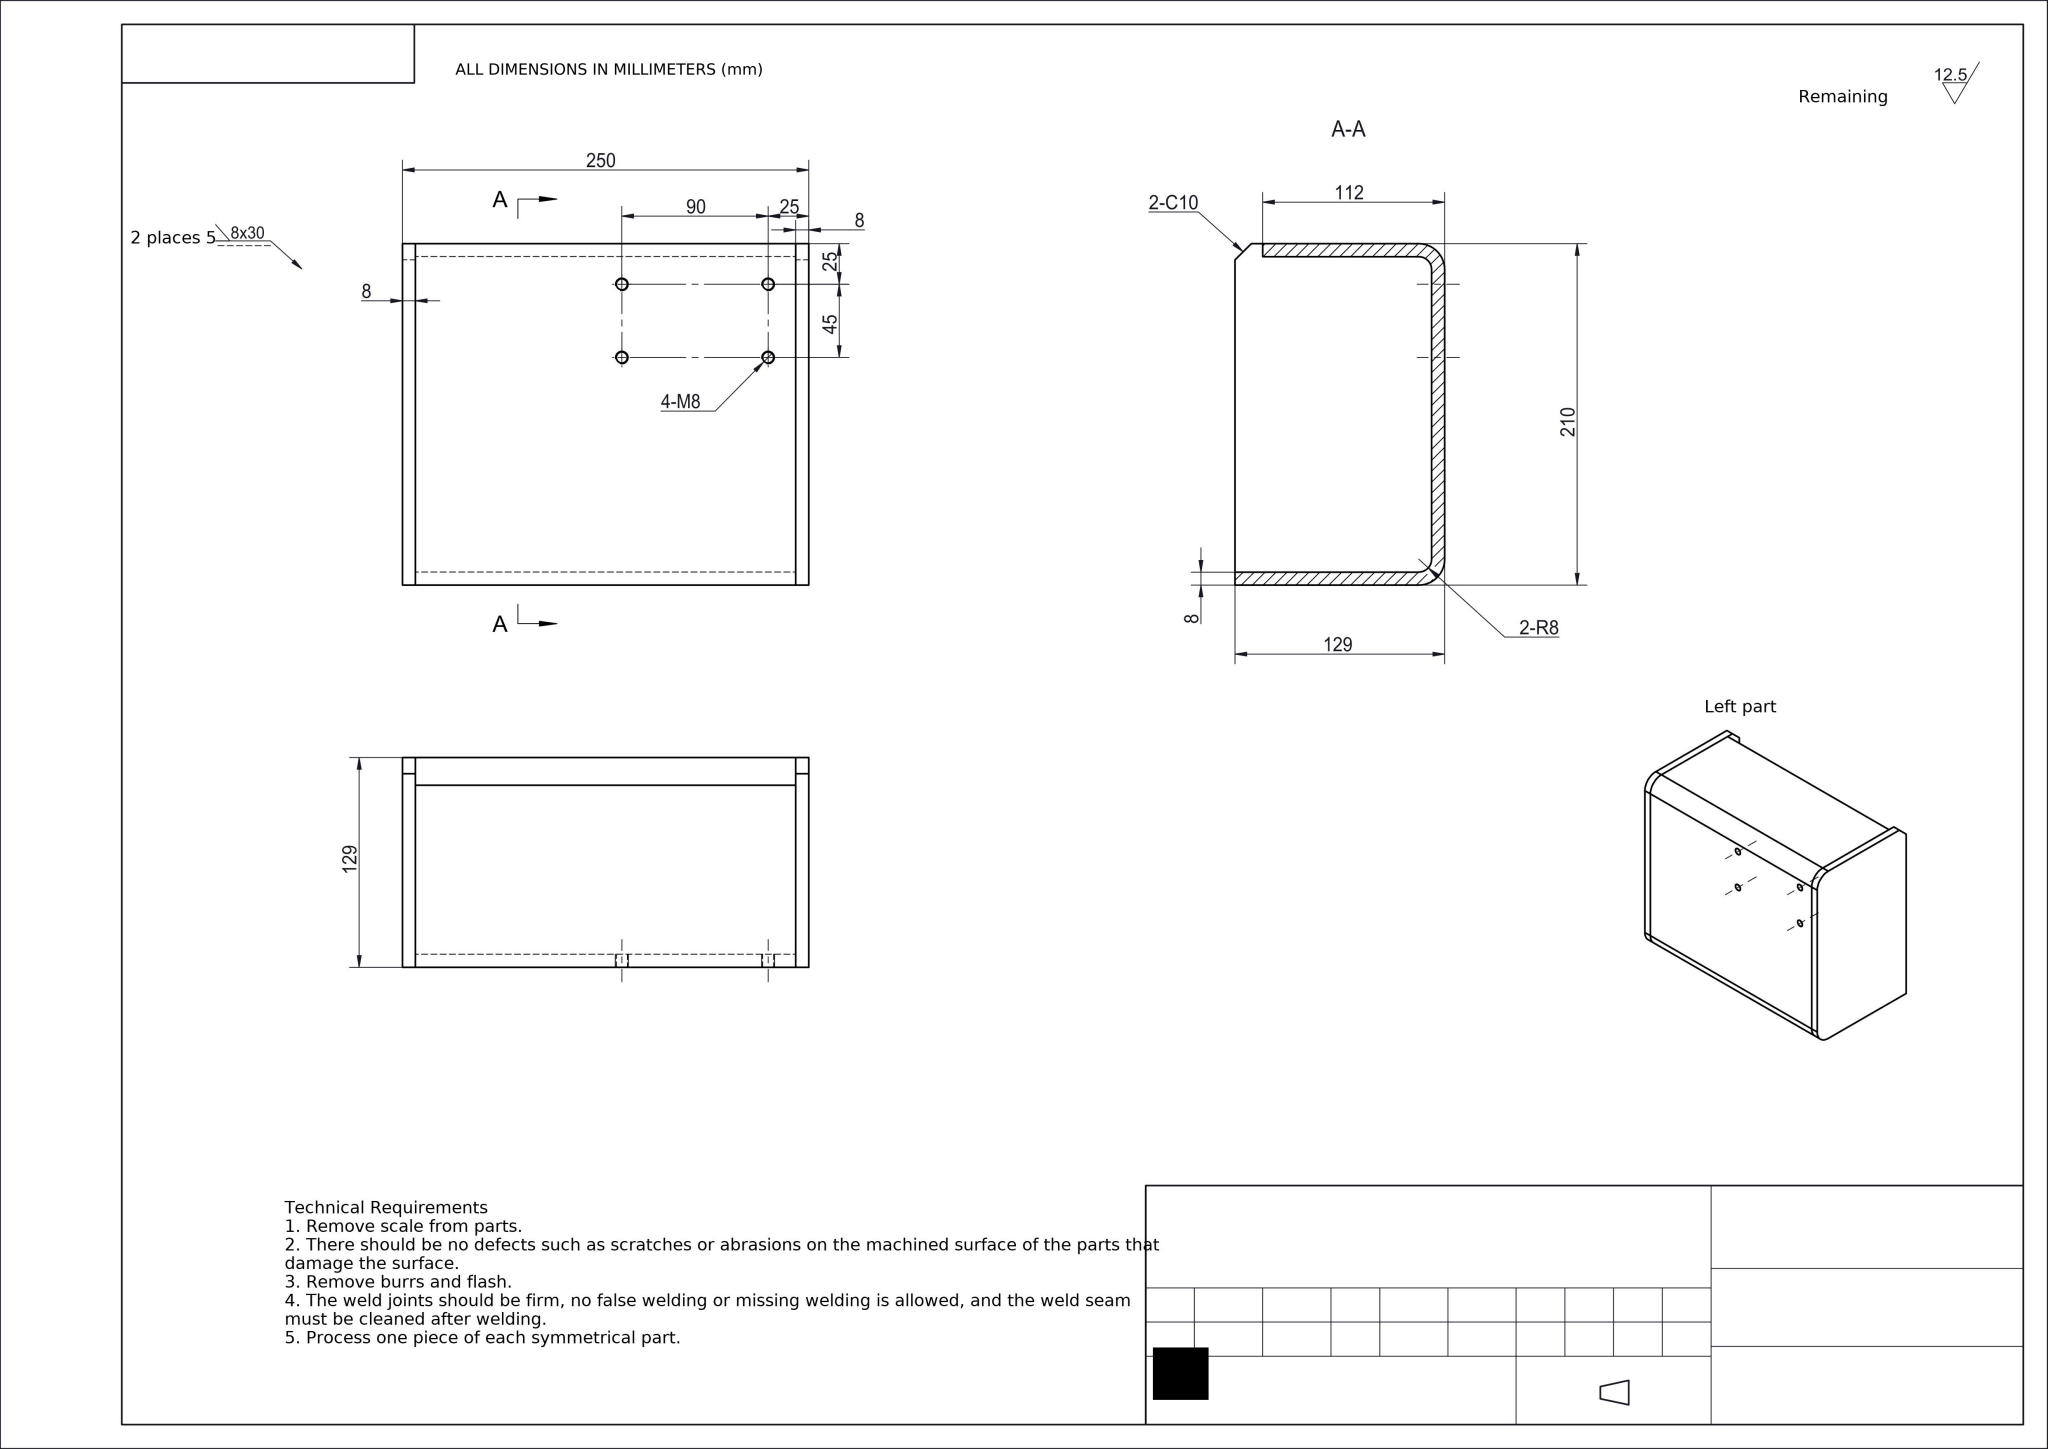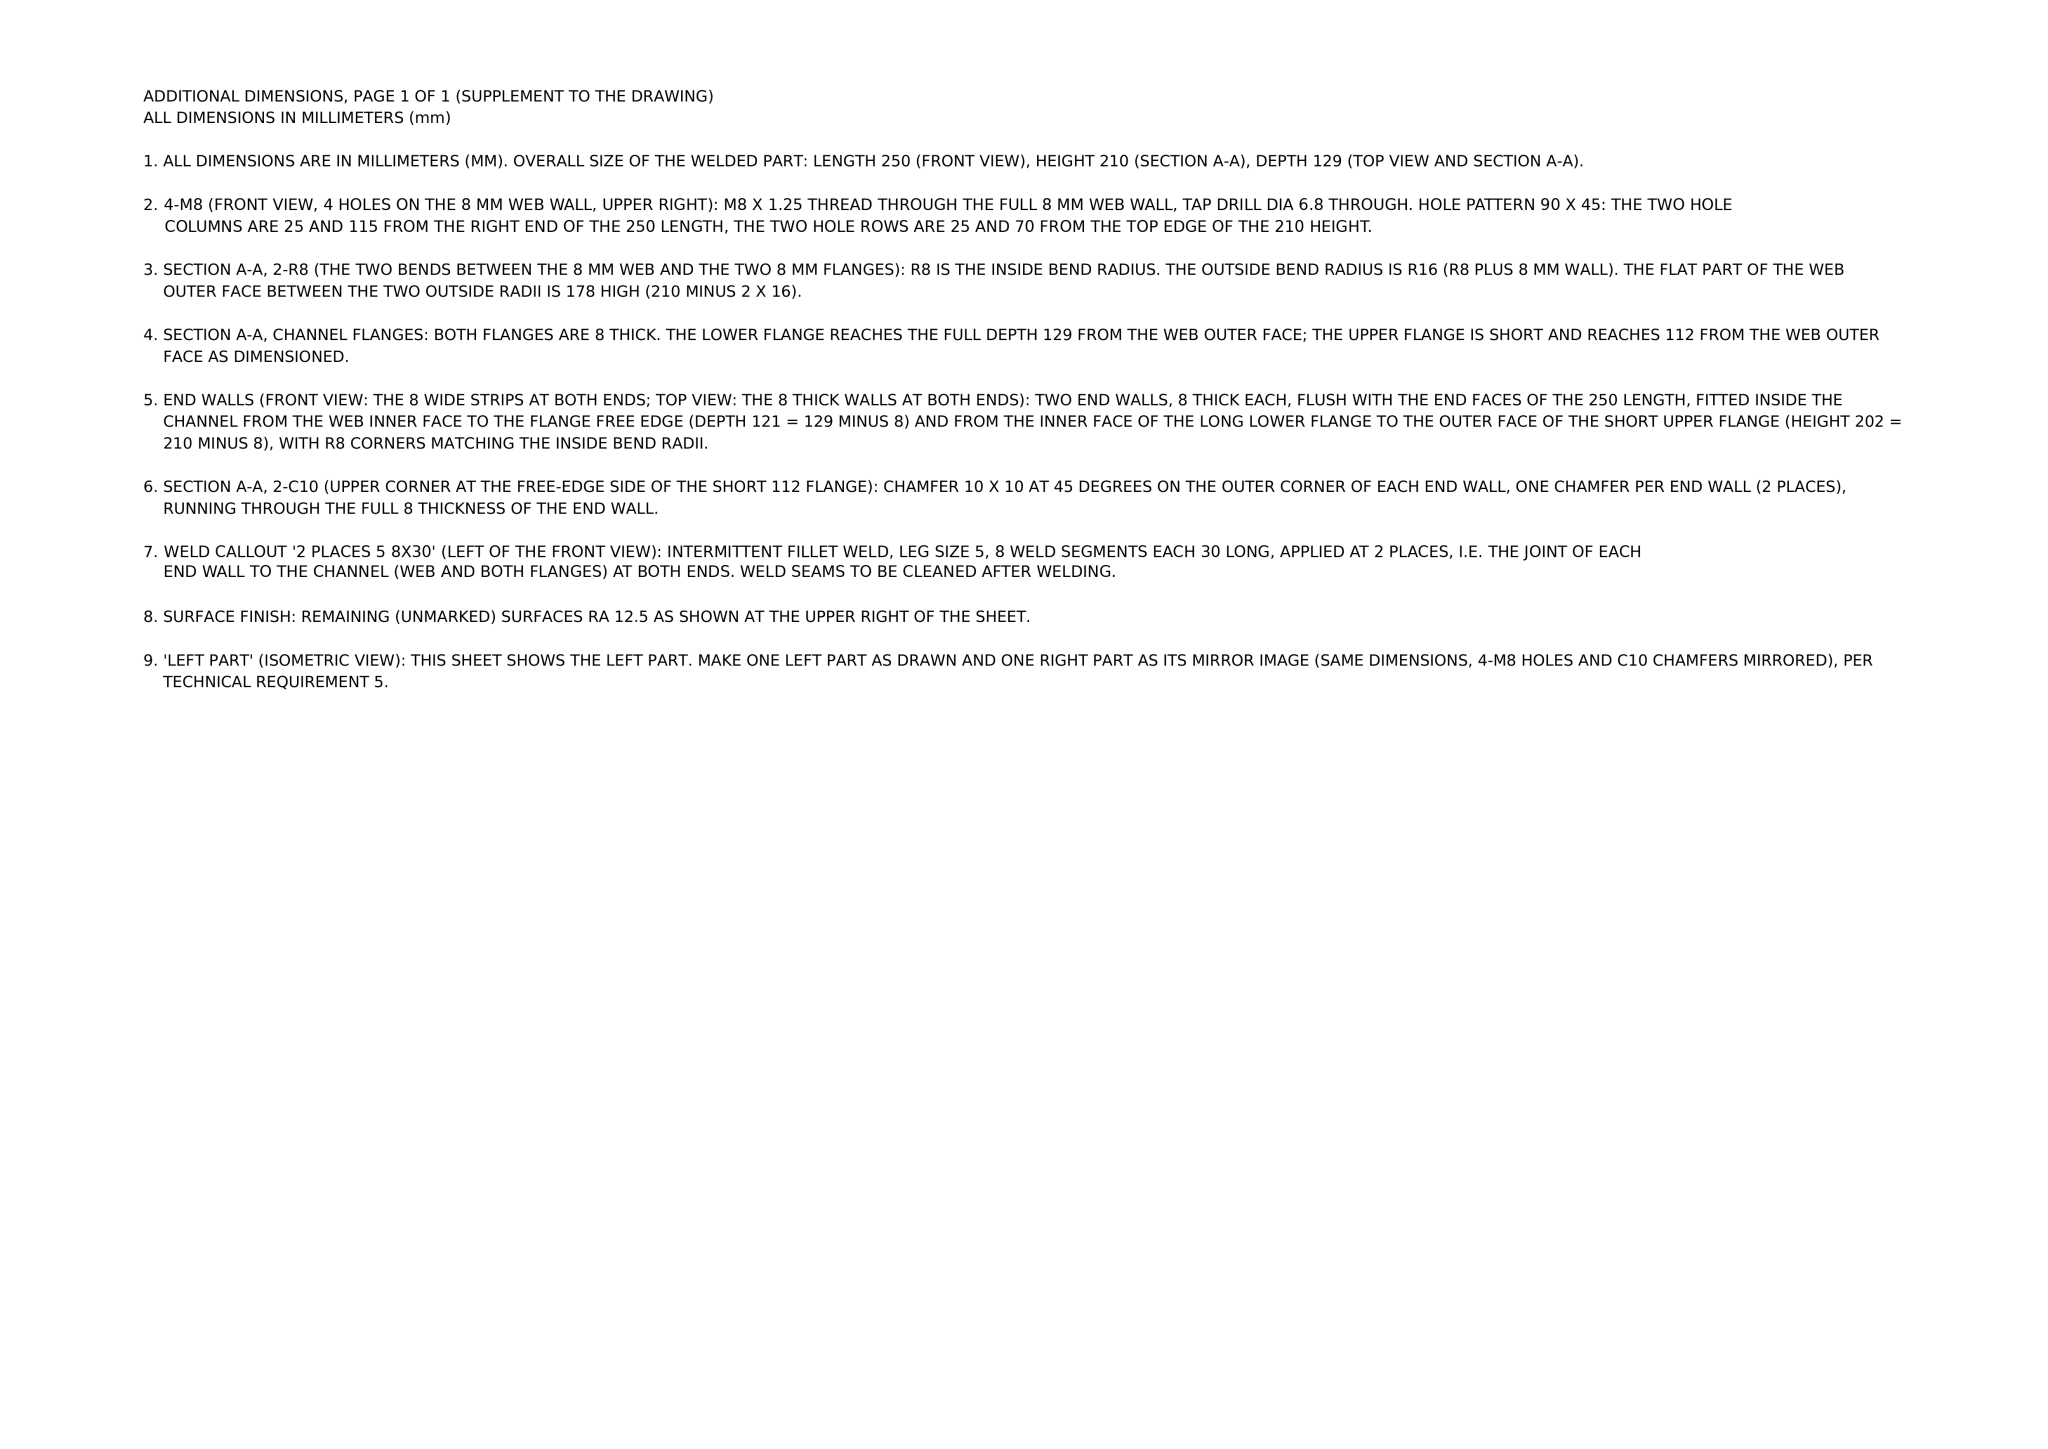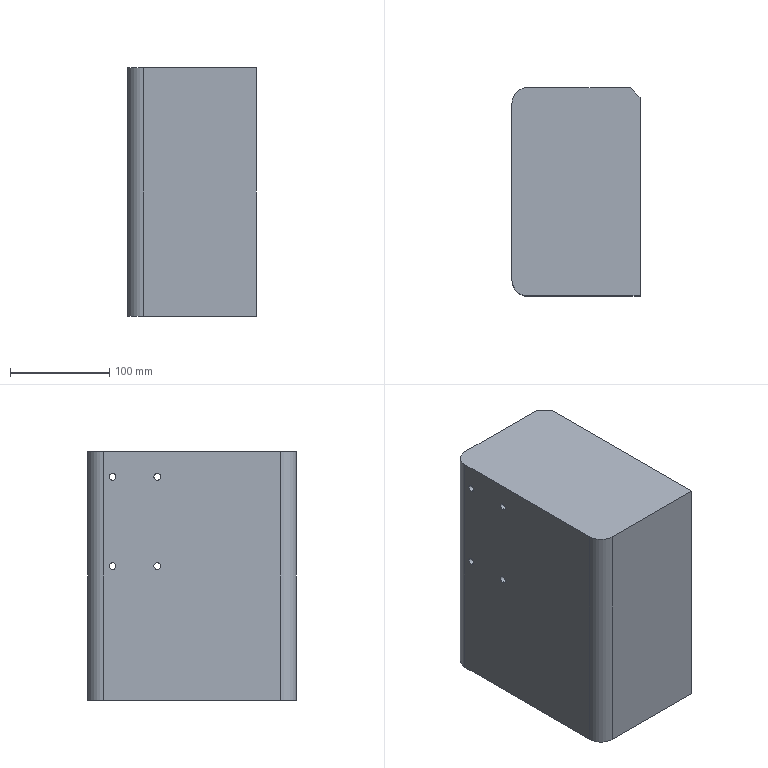Part | NX | mm | 1 solid | 26 faces | box 129 x 210 x 250 mm | volume 1224757 mm3 | plane 14 | cylinder 12 | commonest cylinder face diameters 6.8 x8 32 x2 16 x2
STEP:
#1=COLOUR_RGB('',0.7922,0.8196,0.9333);
#2=FILL_AREA_STYLE_COLOUR('',#1);
#3=FILL_AREA_STYLE('',(#2));
#4=SURFACE_STYLE_FILL_AREA(#3);
#5=SURFACE_SIDE_STYLE('',(#4));
#6=SURFACE_STYLE_USAGE(.BOTH.,#5);
#7=PRESENTATION_STYLE_ASSIGNMENT((#6));
#8=CARTESIAN_POINT('',(8.,80.,6.6));
#9=VERTEX_POINT('',#8);
#10=CARTESIAN_POINT('',(0.,80.,6.6));
#11=VERTEX_POINT('',#10);
#12=CARTESIAN_POINT('',(0.,80.,6.6));
#13=DIRECTION('',(-1.,0.,0.));
#14=VECTOR('',#13,1000.);
#15=LINE('',#12,#14);
#16=EDGE_CURVE('',#9,#11,#15,.T.);
#17=ORIENTED_EDGE('',*,*,#16,.F.);
#18=CARTESIAN_POINT('',(8.,80.,13.4));
#19=VERTEX_POINT('',#18);
#20=CARTESIAN_POINT('',(8.,80.,10.));
#21=DIRECTION('',(1.,0.,0.));
#22=DIRECTION('',(0.,1.,0.));
#23=AXIS2_PLACEMENT_3D('',#20,#21,#22);
#24=CIRCLE('',#23,3.4);
#25=EDGE_CURVE('',#9,#19,#24,.T.);
#26=ORIENTED_EDGE('',*,*,#25,.T.);
#27=CARTESIAN_POINT('',(0.,80.,13.4));
#28=VERTEX_POINT('',#27);
#29=CARTESIAN_POINT('',(0.,80.,13.4));
#30=DIRECTION('',(-1.,0.,0.));
#31=VECTOR('',#30,1000.);
#32=LINE('',#29,#31);
#33=EDGE_CURVE('',#19,#28,#32,.T.);
#34=ORIENTED_EDGE('',*,*,#33,.T.);
#35=CARTESIAN_POINT('',(0.,80.,10.));
#36=DIRECTION('',(-1.,0.,0.));
#37=DIRECTION('',(0.,0.,1.));
#38=AXIS2_PLACEMENT_3D('',#35,#36,#37);
#39=CIRCLE('',#38,3.4);
#40=EDGE_CURVE('',#28,#11,#39,.T.);
#41=ORIENTED_EDGE('',*,*,#40,.T.);
#42=EDGE_LOOP('',(#17,#26,#34,#41));
#43=FACE_OUTER_BOUND('',#42,.T.);
#44=CARTESIAN_POINT('',(0.,80.,10.));
#45=DIRECTION('',(-1.,0.,0.));
#46=DIRECTION('',(0.,0.,1.));
#47=AXIS2_PLACEMENT_3D('',#44,#45,#46);
#48=CYLINDRICAL_SURFACE('',#47,3.4);
#49=ADVANCED_FACE('',(#43),#48,.F.);
#50=CARTESIAN_POINT('',(8.,35.,6.6));
#51=VERTEX_POINT('',#50);
#52=CARTESIAN_POINT('',(-0.,35.,6.6));
#53=VERTEX_POINT('',#52);
#54=CARTESIAN_POINT('',(-0.,35.,6.6));
#55=DIRECTION('',(-1.,0.,0.));
#56=VECTOR('',#55,1000.);
#57=LINE('',#54,#56);
#58=EDGE_CURVE('',#51,#53,#57,.T.);
#59=ORIENTED_EDGE('',*,*,#58,.F.);
#60=CARTESIAN_POINT('',(8.,35.,13.4));
#61=VERTEX_POINT('',#60);
#62=CARTESIAN_POINT('',(8.,35.,10.));
#63=DIRECTION('',(1.,0.,0.));
#64=DIRECTION('',(0.,1.,0.));
#65=AXIS2_PLACEMENT_3D('',#62,#63,#64);
#66=CIRCLE('',#65,3.4);
#67=EDGE_CURVE('',#51,#61,#66,.T.);
#68=ORIENTED_EDGE('',*,*,#67,.T.);
#69=CARTESIAN_POINT('',(-0.,35.,13.4));
#70=VERTEX_POINT('',#69);
#71=CARTESIAN_POINT('',(-0.,35.,13.4));
#72=DIRECTION('',(-1.,0.,0.));
#73=VECTOR('',#72,1000.);
#74=LINE('',#71,#73);
#75=EDGE_CURVE('',#61,#70,#74,.T.);
#76=ORIENTED_EDGE('',*,*,#75,.T.);
#77=CARTESIAN_POINT('',(-0.,35.,10.));
#78=DIRECTION('',(-1.,0.,0.));
#79=DIRECTION('',(0.,0.,1.));
#80=AXIS2_PLACEMENT_3D('',#77,#78,#79);
#81=CIRCLE('',#80,3.4);
#82=EDGE_CURVE('',#70,#53,#81,.T.);
#83=ORIENTED_EDGE('',*,*,#82,.T.);
#84=EDGE_LOOP('',(#59,#68,#76,#83));
#85=FACE_OUTER_BOUND('',#84,.T.);
#86=CARTESIAN_POINT('',(-0.,35.,10.));
#87=DIRECTION('',(-1.,0.,0.));
#88=DIRECTION('',(0.,0.,1.));
#89=AXIS2_PLACEMENT_3D('',#86,#87,#88);
#90=CYLINDRICAL_SURFACE('',#89,3.4);
#91=ADVANCED_FACE('',(#85),#90,.F.);
#92=CARTESIAN_POINT('',(8.,80.,96.6));
#93=VERTEX_POINT('',#92);
#94=CARTESIAN_POINT('',(0.,80.,96.6));
#95=VERTEX_POINT('',#94);
#96=CARTESIAN_POINT('',(0.,80.,96.6));
#97=DIRECTION('',(-1.,0.,0.));
#98=VECTOR('',#97,1000.);
#99=LINE('',#96,#98);
#100=EDGE_CURVE('',#93,#95,#99,.T.);
#101=ORIENTED_EDGE('',*,*,#100,.F.);
#102=CARTESIAN_POINT('',(8.,80.,103.4));
#103=VERTEX_POINT('',#102);
#104=CARTESIAN_POINT('',(8.,80.,100.));
#105=DIRECTION('',(1.,0.,0.));
#106=DIRECTION('',(0.,1.,0.));
#107=AXIS2_PLACEMENT_3D('',#104,#105,#106);
#108=CIRCLE('',#107,3.4);
#109=EDGE_CURVE('',#93,#103,#108,.T.);
#110=ORIENTED_EDGE('',*,*,#109,.T.);
#111=CARTESIAN_POINT('',(0.,80.,103.4));
#112=VERTEX_POINT('',#111);
#113=CARTESIAN_POINT('',(0.,80.,103.4));
#114=DIRECTION('',(-1.,0.,0.));
#115=VECTOR('',#114,1000.);
#116=LINE('',#113,#115);
#117=EDGE_CURVE('',#103,#112,#116,.T.);
#118=ORIENTED_EDGE('',*,*,#117,.T.);
#119=CARTESIAN_POINT('',(0.,80.,100.));
#120=DIRECTION('',(-1.,0.,0.));
#121=DIRECTION('',(0.,0.,1.));
#122=AXIS2_PLACEMENT_3D('',#119,#120,#121);
#123=CIRCLE('',#122,3.4);
#124=EDGE_CURVE('',#112,#95,#123,.T.);
#125=ORIENTED_EDGE('',*,*,#124,.T.);
#126=EDGE_LOOP('',(#101,#110,#118,#125));
#127=FACE_OUTER_BOUND('',#126,.T.);
#128=CARTESIAN_POINT('',(0.,80.,100.));
#129=DIRECTION('',(-1.,0.,0.));
#130=DIRECTION('',(0.,0.,1.));
#131=AXIS2_PLACEMENT_3D('',#128,#129,#130);
#132=CYLINDRICAL_SURFACE('',#131,3.4);
#133=ADVANCED_FACE('',(#127),#132,.F.);
#134=CARTESIAN_POINT('',(8.,35.,96.6));
#135=VERTEX_POINT('',#134);
#136=CARTESIAN_POINT('',(-0.,35.,96.6));
#137=VERTEX_POINT('',#136);
#138=CARTESIAN_POINT('',(-0.,35.,96.6));
#139=DIRECTION('',(-1.,0.,0.));
#140=VECTOR('',#139,1000.);
#141=LINE('',#138,#140);
#142=EDGE_CURVE('',#135,#137,#141,.T.);
#143=ORIENTED_EDGE('',*,*,#142,.F.);
#144=CARTESIAN_POINT('',(8.,35.,103.4));
#145=VERTEX_POINT('',#144);
#146=CARTESIAN_POINT('',(8.,35.,100.));
#147=DIRECTION('',(1.,0.,0.));
#148=DIRECTION('',(0.,1.,0.));
#149=AXIS2_PLACEMENT_3D('',#146,#147,#148);
#150=CIRCLE('',#149,3.4);
#151=EDGE_CURVE('',#135,#145,#150,.T.);
#152=ORIENTED_EDGE('',*,*,#151,.T.);
#153=CARTESIAN_POINT('',(-0.,35.,103.4));
#154=VERTEX_POINT('',#153);
#155=CARTESIAN_POINT('',(-0.,35.,103.4));
#156=DIRECTION('',(-1.,0.,0.));
#157=VECTOR('',#156,1000.);
#158=LINE('',#155,#157);
#159=EDGE_CURVE('',#145,#154,#158,.T.);
#160=ORIENTED_EDGE('',*,*,#159,.T.);
#161=CARTESIAN_POINT('',(-0.,35.,100.));
#162=DIRECTION('',(-1.,0.,0.));
#163=DIRECTION('',(0.,0.,1.));
#164=AXIS2_PLACEMENT_3D('',#161,#162,#163);
#165=CIRCLE('',#164,3.4);
#166=EDGE_CURVE('',#154,#137,#165,.T.);
#167=ORIENTED_EDGE('',*,*,#166,.T.);
#168=EDGE_LOOP('',(#143,#152,#160,#167));
#169=FACE_OUTER_BOUND('',#168,.T.);
#170=CARTESIAN_POINT('',(-0.,35.,100.));
#171=DIRECTION('',(-1.,0.,0.));
#172=DIRECTION('',(0.,0.,1.));
#173=AXIS2_PLACEMENT_3D('',#170,#171,#172);
#174=CYLINDRICAL_SURFACE('',#173,3.4);
#175=ADVANCED_FACE('',(#169),#174,.F.);
#176=CARTESIAN_POINT('',(-0.,-89.,125.));
#177=VERTEX_POINT('',#176);
#178=CARTESIAN_POINT('',(-0.,-89.,-125.));
#179=VERTEX_POINT('',#178);
#180=CARTESIAN_POINT('',(-0.,-89.,117.));
#181=DIRECTION('',(0.,0.,-1.));
#182=VECTOR('',#181,1000.);
#183=LINE('',#180,#182);
#184=EDGE_CURVE('',#177,#179,#183,.T.);
#185=ORIENTED_EDGE('',*,*,#184,.T.);
#186=CARTESIAN_POINT('',(16.,-105.,-125.));
#187=VERTEX_POINT('',#186);
#188=CARTESIAN_POINT('',(16.,-89.,-125.));
#189=DIRECTION('',(0.,-0.,-1.));
#190=DIRECTION('',(-1.,0.,0.));
#191=AXIS2_PLACEMENT_3D('',#188,#189,#190);
#192=CIRCLE('',#191,16.);
#193=EDGE_CURVE('',#187,#179,#192,.T.);
#194=ORIENTED_EDGE('',*,*,#193,.F.);
#195=CARTESIAN_POINT('',(16.,-105.,125.));
#196=VERTEX_POINT('',#195);
#197=CARTESIAN_POINT('',(16.,-105.,117.));
#198=DIRECTION('',(0.,0.,-1.));
#199=VECTOR('',#198,1000.);
#200=LINE('',#197,#199);
#201=EDGE_CURVE('',#196,#187,#200,.T.);
#202=ORIENTED_EDGE('',*,*,#201,.F.);
#203=CARTESIAN_POINT('',(16.,-89.,125.));
#204=DIRECTION('',(0.,0.,1.));
#205=DIRECTION('',(1.,0.,0.));
#206=AXIS2_PLACEMENT_3D('',#203,#204,#205);
#207=CIRCLE('',#206,16.);
#208=EDGE_CURVE('',#177,#196,#207,.T.);
#209=ORIENTED_EDGE('',*,*,#208,.F.);
#210=EDGE_LOOP('',(#185,#194,#202,#209));
#211=FACE_OUTER_BOUND('',#210,.T.);
#212=CARTESIAN_POINT('',(16.,-89.,117.));
#213=DIRECTION('',(0.,0.,-1.));
#214=DIRECTION('',(-1.,0.,0.));
#215=AXIS2_PLACEMENT_3D('',#212,#213,#214);
#216=CYLINDRICAL_SURFACE('',#215,16.);
#217=ADVANCED_FACE('',(#211),#216,.T.);
#218=ORIENTED_EDGE('',*,*,#166,.F.);
#219=CARTESIAN_POINT('',(-0.,35.,100.));
#220=DIRECTION('',(-1.,0.,0.));
#221=DIRECTION('',(0.,0.,1.));
#222=AXIS2_PLACEMENT_3D('',#219,#220,#221);
#223=CIRCLE('',#222,3.4);
#224=EDGE_CURVE('',#137,#154,#223,.T.);
#225=ORIENTED_EDGE('',*,*,#224,.F.);
#226=EDGE_LOOP('',(#218,#225));
#227=FACE_BOUND('',#226,.T.);
#228=ORIENTED_EDGE('',*,*,#124,.F.);
#229=CARTESIAN_POINT('',(0.,80.,100.));
#230=DIRECTION('',(-1.,0.,0.));
#231=DIRECTION('',(0.,0.,1.));
#232=AXIS2_PLACEMENT_3D('',#229,#230,#231);
#233=CIRCLE('',#232,3.4);
#234=EDGE_CURVE('',#95,#112,#233,.T.);
#235=ORIENTED_EDGE('',*,*,#234,.F.);
#236=EDGE_LOOP('',(#228,#235));
#237=FACE_BOUND('',#236,.T.);
#238=ORIENTED_EDGE('',*,*,#82,.F.);
#239=CARTESIAN_POINT('',(-0.,35.,10.));
#240=DIRECTION('',(-1.,0.,0.));
#241=DIRECTION('',(0.,0.,1.));
#242=AXIS2_PLACEMENT_3D('',#239,#240,#241);
#243=CIRCLE('',#242,3.4);
#244=EDGE_CURVE('',#53,#70,#243,.T.);
#245=ORIENTED_EDGE('',*,*,#244,.F.);
#246=EDGE_LOOP('',(#238,#245));
#247=FACE_BOUND('',#246,.T.);
#248=ORIENTED_EDGE('',*,*,#40,.F.);
#249=CARTESIAN_POINT('',(0.,80.,10.));
#250=DIRECTION('',(-1.,0.,0.));
#251=DIRECTION('',(0.,0.,1.));
#252=AXIS2_PLACEMENT_3D('',#249,#250,#251);
#253=CIRCLE('',#252,3.4);
#254=EDGE_CURVE('',#11,#28,#253,.T.);
#255=ORIENTED_EDGE('',*,*,#254,.F.);
#256=EDGE_LOOP('',(#248,#255));
#257=FACE_BOUND('',#256,.T.);
#258=CARTESIAN_POINT('',(0.,89.,125.));
#259=VERTEX_POINT('',#258);
#260=CARTESIAN_POINT('',(0.,89.,-125.));
#261=VERTEX_POINT('',#260);
#262=CARTESIAN_POINT('',(0.,89.,117.));
#263=DIRECTION('',(0.,0.,-1.));
#264=VECTOR('',#263,1000.);
#265=LINE('',#262,#264);
#266=EDGE_CURVE('',#259,#261,#265,.T.);
#267=ORIENTED_EDGE('',*,*,#266,.T.);
#268=CARTESIAN_POINT('',(-0.,105.,-125.));
#269=DIRECTION('',(-0.,-1.,-0.));
#270=VECTOR('',#269,1000.);
#271=LINE('',#268,#270);
#272=EDGE_CURVE('',#261,#179,#271,.T.);
#273=ORIENTED_EDGE('',*,*,#272,.T.);
#274=ORIENTED_EDGE('',*,*,#184,.F.);
#275=CARTESIAN_POINT('',(-0.,105.,125.));
#276=DIRECTION('',(0.,-1.,-0.));
#277=VECTOR('',#276,1000.);
#278=LINE('',#275,#277);
#279=EDGE_CURVE('',#259,#177,#278,.T.);
#280=ORIENTED_EDGE('',*,*,#279,.F.);
#281=EDGE_LOOP('',(#267,#273,#274,#280));
#282=FACE_OUTER_BOUND('',#281,.T.);
#283=CARTESIAN_POINT('',(-0.,105.,117.));
#284=DIRECTION('',(1.,0.,0.));
#285=DIRECTION('',(0.,1.,0.));
#286=AXIS2_PLACEMENT_3D('',#283,#284,#285);
#287=PLANE('',#286);
#288=ADVANCED_FACE('',(#227,#237,#247,#257,#282),#287,.F.);
#289=CARTESIAN_POINT('',(16.,105.,125.));
#290=VERTEX_POINT('',#289);
#291=CARTESIAN_POINT('',(16.,105.,-125.));
#292=VERTEX_POINT('',#291);
#293=CARTESIAN_POINT('',(16.,105.,117.));
#294=DIRECTION('',(0.,0.,-1.));
#295=VECTOR('',#294,1000.);
#296=LINE('',#293,#295);
#297=EDGE_CURVE('',#290,#292,#296,.T.);
#298=ORIENTED_EDGE('',*,*,#297,.T.);
#299=CARTESIAN_POINT('',(16.,89.,-125.));
#300=DIRECTION('',(0.,-0.,-1.));
#301=DIRECTION('',(-1.,0.,0.));
#302=AXIS2_PLACEMENT_3D('',#299,#300,#301);
#303=CIRCLE('',#302,16.);
#304=EDGE_CURVE('',#261,#292,#303,.T.);
#305=ORIENTED_EDGE('',*,*,#304,.F.);
#306=ORIENTED_EDGE('',*,*,#266,.F.);
#307=CARTESIAN_POINT('',(16.,89.,125.));
#308=DIRECTION('',(0.,0.,1.));
#309=DIRECTION('',(1.,0.,0.));
#310=AXIS2_PLACEMENT_3D('',#307,#308,#309);
#311=CIRCLE('',#310,16.);
#312=EDGE_CURVE('',#290,#259,#311,.T.);
#313=ORIENTED_EDGE('',*,*,#312,.F.);
#314=EDGE_LOOP('',(#298,#305,#306,#313));
#315=FACE_OUTER_BOUND('',#314,.T.);
#316=CARTESIAN_POINT('',(16.,89.,117.));
#317=DIRECTION('',(0.,0.,-1.));
#318=DIRECTION('',(-1.,0.,0.));
#319=AXIS2_PLACEMENT_3D('',#316,#317,#318);
#320=CYLINDRICAL_SURFACE('',#319,16.);
#321=ADVANCED_FACE('',(#315),#320,.T.);
#322=CARTESIAN_POINT('',(112.,105.,117.));
#323=VERTEX_POINT('',#322);
#324=CARTESIAN_POINT('',(112.,105.,-117.));
#325=VERTEX_POINT('',#324);
#326=CARTESIAN_POINT('',(112.,105.,117.));
#327=DIRECTION('',(0.,0.,-1.));
#328=VECTOR('',#327,1000.);
#329=LINE('',#326,#328);
#330=EDGE_CURVE('',#323,#325,#329,.T.);
#331=ORIENTED_EDGE('',*,*,#330,.T.);
#332=CARTESIAN_POINT('',(119.,105.,-117.));
#333=VERTEX_POINT('',#332);
#334=CARTESIAN_POINT('',(112.,105.,-117.));
#335=DIRECTION('',(-1.,-0.,-0.));
#336=VECTOR('',#335,1000.);
#337=LINE('',#334,#336);
#338=EDGE_CURVE('',#333,#325,#337,.T.);
#339=ORIENTED_EDGE('',*,*,#338,.F.);
#340=CARTESIAN_POINT('',(119.,105.,-125.));
#341=VERTEX_POINT('',#340);
#342=CARTESIAN_POINT('',(119.,105.,-125.));
#343=DIRECTION('',(-0.,-0.,-1.));
#344=VECTOR('',#343,1000.);
#345=LINE('',#342,#344);
#346=EDGE_CURVE('',#333,#341,#345,.T.);
#347=ORIENTED_EDGE('',*,*,#346,.T.);
#348=CARTESIAN_POINT('',(129.,105.,-125.));
#349=DIRECTION('',(-1.,-0.,-0.));
#350=VECTOR('',#349,1000.);
#351=LINE('',#348,#350);
#352=EDGE_CURVE('',#341,#292,#351,.T.);
#353=ORIENTED_EDGE('',*,*,#352,.T.);
#354=ORIENTED_EDGE('',*,*,#297,.F.);
#355=CARTESIAN_POINT('',(119.,105.,125.));
#356=VERTEX_POINT('',#355);
#357=CARTESIAN_POINT('',(129.,105.,125.));
#358=DIRECTION('',(-1.,0.,0.));
#359=VECTOR('',#358,1000.);
#360=LINE('',#357,#359);
#361=EDGE_CURVE('',#356,#290,#360,.T.);
#362=ORIENTED_EDGE('',*,*,#361,.F.);
#363=CARTESIAN_POINT('',(119.,105.,117.));
#364=VERTEX_POINT('',#363);
#365=CARTESIAN_POINT('',(119.,105.,125.));
#366=DIRECTION('',(0.,-0.,-1.));
#367=VECTOR('',#366,1000.);
#368=LINE('',#365,#367);
#369=EDGE_CURVE('',#356,#364,#368,.T.);
#370=ORIENTED_EDGE('',*,*,#369,.T.);
#371=CARTESIAN_POINT('',(112.,105.,117.));
#372=DIRECTION('',(-1.,0.,0.));
#373=VECTOR('',#372,1000.);
#374=LINE('',#371,#373);
#375=EDGE_CURVE('',#364,#323,#374,.T.);
#376=ORIENTED_EDGE('',*,*,#375,.T.);
#377=EDGE_LOOP('',(#331,#339,#347,#353,#354,#362,#370,#376));
#378=FACE_OUTER_BOUND('',#377,.T.);
#379=CARTESIAN_POINT('',(112.,105.,117.));
#380=DIRECTION('',(0.,-1.,0.));
#381=DIRECTION('',(0.,0.,-1.));
#382=AXIS2_PLACEMENT_3D('',#379,#380,#381);
#383=PLANE('',#382);
#384=ADVANCED_FACE('',(#378),#383,.F.);
#385=CARTESIAN_POINT('',(112.,97.,-117.));
#386=VERTEX_POINT('',#385);
#387=CARTESIAN_POINT('',(112.,105.,-117.));
#388=DIRECTION('',(0.,-1.,0.));
#389=VECTOR('',#388,1000.);
#390=LINE('',#387,#389);
#391=EDGE_CURVE('',#325,#386,#390,.T.);
#392=ORIENTED_EDGE('',*,*,#391,.F.);
#393=ORIENTED_EDGE('',*,*,#330,.F.);
#394=CARTESIAN_POINT('',(112.,97.,117.));
#395=VERTEX_POINT('',#394);
#396=CARTESIAN_POINT('',(112.,105.,117.));
#397=DIRECTION('',(0.,-1.,0.));
#398=VECTOR('',#397,1000.);
#399=LINE('',#396,#398);
#400=EDGE_CURVE('',#323,#395,#399,.T.);
#401=ORIENTED_EDGE('',*,*,#400,.T.);
#402=CARTESIAN_POINT('',(112.,97.,117.));
#403=DIRECTION('',(0.,0.,-1.));
#404=VECTOR('',#403,1000.);
#405=LINE('',#402,#404);
#406=EDGE_CURVE('',#395,#386,#405,.T.);
#407=ORIENTED_EDGE('',*,*,#406,.T.);
#408=EDGE_LOOP('',(#392,#393,#401,#407));
#409=FACE_OUTER_BOUND('',#408,.T.);
#410=CARTESIAN_POINT('',(112.,105.,117.));
#411=DIRECTION('',(1.,0.,0.));
#412=DIRECTION('',(0.,1.,0.));
#413=AXIS2_PLACEMENT_3D('',#410,#411,#412);
#414=PLANE('',#413);
#415=ADVANCED_FACE('',(#409),#414,.T.);
#416=CARTESIAN_POINT('',(16.,97.,-117.));
#417=VERTEX_POINT('',#416);
#418=CARTESIAN_POINT('',(112.,97.,-117.));
#419=DIRECTION('',(-1.,-0.,0.));
#420=VECTOR('',#419,1000.);
#421=LINE('',#418,#420);
#422=EDGE_CURVE('',#386,#417,#421,.T.);
#423=ORIENTED_EDGE('',*,*,#422,.F.);
#424=ORIENTED_EDGE('',*,*,#406,.F.);
#425=CARTESIAN_POINT('',(16.,97.,117.));
#426=VERTEX_POINT('',#425);
#427=CARTESIAN_POINT('',(112.,97.,117.));
#428=DIRECTION('',(-1.,-0.,0.));
#429=VECTOR('',#428,1000.);
#430=LINE('',#427,#429);
#431=EDGE_CURVE('',#395,#426,#430,.T.);
#432=ORIENTED_EDGE('',*,*,#431,.T.);
#433=CARTESIAN_POINT('',(16.,97.,117.));
#434=DIRECTION('',(0.,0.,-1.));
#435=VECTOR('',#434,1000.);
#436=LINE('',#433,#435);
#437=EDGE_CURVE('',#426,#417,#436,.T.);
#438=ORIENTED_EDGE('',*,*,#437,.T.);
#439=EDGE_LOOP('',(#423,#424,#432,#438));
#440=FACE_OUTER_BOUND('',#439,.T.);
#441=CARTESIAN_POINT('',(112.,97.,117.));
#442=DIRECTION('',(0.,-1.,0.));
#443=DIRECTION('',(0.,0.,-1.));
#444=AXIS2_PLACEMENT_3D('',#441,#442,#443);
#445=PLANE('',#444);
#446=ADVANCED_FACE('',(#440),#445,.T.);
#447=CARTESIAN_POINT('',(8.,89.,-117.));
#448=VERTEX_POINT('',#447);
#449=CARTESIAN_POINT('',(16.,89.,-117.));
#450=DIRECTION('',(0.,0.,1.));
#451=DIRECTION('',(1.,0.,0.));
#452=AXIS2_PLACEMENT_3D('',#449,#450,#451);
#453=CIRCLE('',#452,8.);
#454=EDGE_CURVE('',#417,#448,#453,.T.);
#455=ORIENTED_EDGE('',*,*,#454,.F.);
#456=ORIENTED_EDGE('',*,*,#437,.F.);
#457=CARTESIAN_POINT('',(8.,89.,117.));
#458=VERTEX_POINT('',#457);
#459=CARTESIAN_POINT('',(16.,89.,117.));
#460=DIRECTION('',(0.,0.,1.));
#461=DIRECTION('',(1.,0.,0.));
#462=AXIS2_PLACEMENT_3D('',#459,#460,#461);
#463=CIRCLE('',#462,8.);
#464=EDGE_CURVE('',#426,#458,#463,.T.);
#465=ORIENTED_EDGE('',*,*,#464,.T.);
#466=CARTESIAN_POINT('',(8.,89.,117.));
#467=DIRECTION('',(0.,0.,-1.));
#468=VECTOR('',#467,1000.);
#469=LINE('',#466,#468);
#470=EDGE_CURVE('',#458,#448,#469,.T.);
#471=ORIENTED_EDGE('',*,*,#470,.T.);
#472=EDGE_LOOP('',(#455,#456,#465,#471));
#473=FACE_OUTER_BOUND('',#472,.T.);
#474=CARTESIAN_POINT('',(16.,89.,117.));
#475=DIRECTION('',(0.,0.,-1.));
#476=DIRECTION('',(-1.,0.,0.));
#477=AXIS2_PLACEMENT_3D('',#474,#475,#476);
#478=CYLINDRICAL_SURFACE('',#477,8.);
#479=ADVANCED_FACE('',(#473),#478,.F.);
#480=CARTESIAN_POINT('',(8.,35.,100.));
#481=DIRECTION('',(1.,0.,0.));
#482=DIRECTION('',(0.,1.,0.));
#483=AXIS2_PLACEMENT_3D('',#480,#481,#482);
#484=CIRCLE('',#483,3.4);
#485=EDGE_CURVE('',#145,#135,#484,.T.);
#486=ORIENTED_EDGE('',*,*,#485,.F.);
#487=ORIENTED_EDGE('',*,*,#151,.F.);
#488=EDGE_LOOP('',(#486,#487));
#489=FACE_BOUND('',#488,.T.);
#490=CARTESIAN_POINT('',(8.,80.,100.));
#491=DIRECTION('',(1.,0.,0.));
#492=DIRECTION('',(0.,1.,0.));
#493=AXIS2_PLACEMENT_3D('',#490,#491,#492);
#494=CIRCLE('',#493,3.4);
#495=EDGE_CURVE('',#103,#93,#494,.T.);
#496=ORIENTED_EDGE('',*,*,#495,.F.);
#497=ORIENTED_EDGE('',*,*,#109,.F.);
#498=EDGE_LOOP('',(#496,#497));
#499=FACE_BOUND('',#498,.T.);
#500=CARTESIAN_POINT('',(8.,35.,10.));
#501=DIRECTION('',(1.,0.,0.));
#502=DIRECTION('',(0.,1.,0.));
#503=AXIS2_PLACEMENT_3D('',#500,#501,#502);
#504=CIRCLE('',#503,3.4);
#505=EDGE_CURVE('',#61,#51,#504,.T.);
#506=ORIENTED_EDGE('',*,*,#505,.F.);
#507=ORIENTED_EDGE('',*,*,#67,.F.);
#508=EDGE_LOOP('',(#506,#507));
#509=FACE_BOUND('',#508,.T.);
#510=CARTESIAN_POINT('',(8.,80.,10.));
#511=DIRECTION('',(1.,0.,0.));
#512=DIRECTION('',(0.,1.,0.));
#513=AXIS2_PLACEMENT_3D('',#510,#511,#512);
#514=CIRCLE('',#513,3.4);
#515=EDGE_CURVE('',#19,#9,#514,.T.);
#516=ORIENTED_EDGE('',*,*,#515,.F.);
#517=ORIENTED_EDGE('',*,*,#25,.F.);
#518=EDGE_LOOP('',(#516,#517));
#519=FACE_BOUND('',#518,.T.);
#520=CARTESIAN_POINT('',(8.,-89.,-117.));
#521=VERTEX_POINT('',#520);
#522=CARTESIAN_POINT('',(8.,105.,-117.));
#523=DIRECTION('',(0.,-1.,0.));
#524=VECTOR('',#523,1000.);
#525=LINE('',#522,#524);
#526=EDGE_CURVE('',#448,#521,#525,.T.);
#527=ORIENTED_EDGE('',*,*,#526,.F.);
#528=ORIENTED_EDGE('',*,*,#470,.F.);
#529=CARTESIAN_POINT('',(8.,-89.,117.));
#530=VERTEX_POINT('',#529);
#531=CARTESIAN_POINT('',(8.,105.,117.));
#532=DIRECTION('',(0.,-1.,0.));
#533=VECTOR('',#532,1000.);
#534=LINE('',#531,#533);
#535=EDGE_CURVE('',#458,#530,#534,.T.);
#536=ORIENTED_EDGE('',*,*,#535,.T.);
#537=CARTESIAN_POINT('',(8.,-89.,117.));
#538=DIRECTION('',(0.,0.,-1.));
#539=VECTOR('',#538,1000.);
#540=LINE('',#537,#539);
#541=EDGE_CURVE('',#530,#521,#540,.T.);
#542=ORIENTED_EDGE('',*,*,#541,.T.);
#543=EDGE_LOOP('',(#527,#528,#536,#542));
#544=FACE_OUTER_BOUND('',#543,.T.);
#545=CARTESIAN_POINT('',(8.,105.,117.));
#546=DIRECTION('',(1.,0.,0.));
#547=DIRECTION('',(0.,1.,0.));
#548=AXIS2_PLACEMENT_3D('',#545,#546,#547);
#549=PLANE('',#548);
#550=ADVANCED_FACE('',(#489,#499,#509,#519,#544),#549,.T.);
#551=CARTESIAN_POINT('',(16.,-97.,-117.));
#552=VERTEX_POINT('',#551);
#553=CARTESIAN_POINT('',(16.,-89.,-117.));
#554=DIRECTION('',(0.,0.,1.));
#555=DIRECTION('',(1.,0.,0.));
#556=AXIS2_PLACEMENT_3D('',#553,#554,#555);
#557=CIRCLE('',#556,8.);
#558=EDGE_CURVE('',#521,#552,#557,.T.);
#559=ORIENTED_EDGE('',*,*,#558,.F.);
#560=ORIENTED_EDGE('',*,*,#541,.F.);
#561=CARTESIAN_POINT('',(16.,-97.,117.));
#562=VERTEX_POINT('',#561);
#563=CARTESIAN_POINT('',(16.,-89.,117.));
#564=DIRECTION('',(0.,0.,1.));
#565=DIRECTION('',(1.,0.,0.));
#566=AXIS2_PLACEMENT_3D('',#563,#564,#565);
#567=CIRCLE('',#566,8.);
#568=EDGE_CURVE('',#530,#562,#567,.T.);
#569=ORIENTED_EDGE('',*,*,#568,.T.);
#570=CARTESIAN_POINT('',(16.,-97.,117.));
#571=DIRECTION('',(0.,0.,-1.));
#572=VECTOR('',#571,1000.);
#573=LINE('',#570,#572);
#574=EDGE_CURVE('',#562,#552,#573,.T.);
#575=ORIENTED_EDGE('',*,*,#574,.T.);
#576=EDGE_LOOP('',(#559,#560,#569,#575));
#577=FACE_OUTER_BOUND('',#576,.T.);
#578=CARTESIAN_POINT('',(16.,-89.,117.));
#579=DIRECTION('',(0.,0.,-1.));
#580=DIRECTION('',(-1.,0.,0.));
#581=AXIS2_PLACEMENT_3D('',#578,#579,#580);
#582=CYLINDRICAL_SURFACE('',#581,8.);
#583=ADVANCED_FACE('',(#577),#582,.F.);
#584=CARTESIAN_POINT('',(129.,-97.,-117.));
#585=VERTEX_POINT('',#584);
#586=CARTESIAN_POINT('',(-0.,-97.,-117.));
#587=DIRECTION('',(1.,0.,0.));
#588=VECTOR('',#587,1000.);
#589=LINE('',#586,#588);
#590=EDGE_CURVE('',#552,#585,#589,.T.);
#591=ORIENTED_EDGE('',*,*,#590,.F.);
#592=ORIENTED_EDGE('',*,*,#574,.F.);
#593=CARTESIAN_POINT('',(129.,-97.,117.));
#594=VERTEX_POINT('',#593);
#595=CARTESIAN_POINT('',(-0.,-97.,117.));
#596=DIRECTION('',(1.,0.,0.));
#597=VECTOR('',#596,1000.);
#598=LINE('',#595,#597);
#599=EDGE_CURVE('',#562,#594,#598,.T.);
#600=ORIENTED_EDGE('',*,*,#599,.T.);
#601=CARTESIAN_POINT('',(129.,-97.,117.));
#602=DIRECTION('',(0.,0.,-1.));
#603=VECTOR('',#602,1000.);
#604=LINE('',#601,#603);
#605=EDGE_CURVE('',#594,#585,#604,.T.);
#606=ORIENTED_EDGE('',*,*,#605,.T.);
#607=EDGE_LOOP('',(#591,#592,#600,#606));
#608=FACE_OUTER_BOUND('',#607,.T.);
#609=CARTESIAN_POINT('',(-0.,-97.,117.));
#610=DIRECTION('',(0.,1.,0.));
#611=DIRECTION('',(1.,0.,0.));
#612=AXIS2_PLACEMENT_3D('',#609,#610,#611);
#613=PLANE('',#612);
#614=ADVANCED_FACE('',(#608),#613,.T.);
#615=CARTESIAN_POINT('',(129.,-105.,125.));
#616=VERTEX_POINT('',#615);
#617=CARTESIAN_POINT('',(129.,-105.,-125.));
#618=VERTEX_POINT('',#617);
#619=CARTESIAN_POINT('',(129.,-105.,117.));
#620=DIRECTION('',(0.,0.,-1.));
#621=VECTOR('',#620,1000.);
#622=LINE('',#619,#621);
#623=EDGE_CURVE('',#616,#618,#622,.T.);
#624=ORIENTED_EDGE('',*,*,#623,.T.);
#625=CARTESIAN_POINT('',(129.,95.,-125.));
#626=VERTEX_POINT('',#625);
#627=CARTESIAN_POINT('',(129.,-105.,-125.));
#628=DIRECTION('',(0.,1.,0.));
#629=VECTOR('',#628,1000.);
#630=LINE('',#627,#629);
#631=EDGE_CURVE('',#618,#626,#630,.T.);
#632=ORIENTED_EDGE('',*,*,#631,.T.);
#633=CARTESIAN_POINT('',(129.,95.,-117.));
#634=VERTEX_POINT('',#633);
#635=CARTESIAN_POINT('',(129.,95.,-125.));
#636=DIRECTION('',(0.,0.,1.));
#637=VECTOR('',#636,1000.);
#638=LINE('',#635,#637);
#639=EDGE_CURVE('',#626,#634,#638,.T.);
#640=ORIENTED_EDGE('',*,*,#639,.T.);
#641=CARTESIAN_POINT('',(129.,-105.,-117.));
#642=DIRECTION('',(0.,1.,0.));
#643=VECTOR('',#642,1000.);
#644=LINE('',#641,#643);
#645=EDGE_CURVE('',#585,#634,#644,.T.);
#646=ORIENTED_EDGE('',*,*,#645,.F.);
#647=ORIENTED_EDGE('',*,*,#605,.F.);
#648=CARTESIAN_POINT('',(129.,95.,117.));
#649=VERTEX_POINT('',#648);
#650=CARTESIAN_POINT('',(129.,-105.,117.));
#651=DIRECTION('',(-0.,1.,0.));
#652=VECTOR('',#651,1000.);
#653=LINE('',#650,#652);
#654=EDGE_CURVE('',#594,#649,#653,.T.);
#655=ORIENTED_EDGE('',*,*,#654,.T.);
#656=CARTESIAN_POINT('',(129.,95.,125.));
#657=VERTEX_POINT('',#656);
#658=CARTESIAN_POINT('',(129.,95.,125.));
#659=DIRECTION('',(-0.,0.,1.));
#660=VECTOR('',#659,1000.);
#661=LINE('',#658,#660);
#662=EDGE_CURVE('',#649,#657,#661,.T.);
#663=ORIENTED_EDGE('',*,*,#662,.T.);
#664=CARTESIAN_POINT('',(129.,-105.,125.));
#665=DIRECTION('',(-0.,1.,0.));
#666=VECTOR('',#665,1000.);
#667=LINE('',#664,#666);
#668=EDGE_CURVE('',#616,#657,#667,.T.);
#669=ORIENTED_EDGE('',*,*,#668,.F.);
#670=EDGE_LOOP('',(#624,#632,#640,#646,#647,#655,#663,#669));
#671=FACE_OUTER_BOUND('',#670,.T.);
#672=CARTESIAN_POINT('',(129.,-97.,117.));
#673=DIRECTION('',(1.,0.,0.));
#674=DIRECTION('',(0.,1.,0.));
#675=AXIS2_PLACEMENT_3D('',#672,#673,#674);
#676=PLANE('',#675);
#677=ADVANCED_FACE('',(#671),#676,.T.);
#678=ORIENTED_EDGE('',*,*,#201,.T.);
#679=CARTESIAN_POINT('',(0.,-105.,-125.));
#680=DIRECTION('',(1.,0.,0.));
#681=VECTOR('',#680,1000.);
#682=LINE('',#679,#681);
#683=EDGE_CURVE('',#187,#618,#682,.T.);
#684=ORIENTED_EDGE('',*,*,#683,.T.);
#685=ORIENTED_EDGE('',*,*,#623,.F.);
#686=CARTESIAN_POINT('',(0.,-105.,125.));
#687=DIRECTION('',(1.,-0.,-0.));
#688=VECTOR('',#687,1000.);
#689=LINE('',#686,#688);
#690=EDGE_CURVE('',#196,#616,#689,.T.);
#691=ORIENTED_EDGE('',*,*,#690,.F.);
#692=EDGE_LOOP('',(#678,#684,#685,#691));
#693=FACE_OUTER_BOUND('',#692,.T.);
#694=CARTESIAN_POINT('',(0.,-105.,117.));
#695=DIRECTION('',(0.,1.,0.));
#696=DIRECTION('',(1.,0.,0.));
#697=AXIS2_PLACEMENT_3D('',#694,#695,#696);
#698=PLANE('',#697);
#699=ADVANCED_FACE('',(#693),#698,.F.);
#700=ORIENTED_EDGE('',*,*,#485,.T.);
#701=ORIENTED_EDGE('',*,*,#142,.T.);
#702=ORIENTED_EDGE('',*,*,#224,.T.);
#703=ORIENTED_EDGE('',*,*,#159,.F.);
#704=EDGE_LOOP('',(#700,#701,#702,#703));
#705=FACE_OUTER_BOUND('',#704,.T.);
#706=CARTESIAN_POINT('',(-0.,35.,100.));
#707=DIRECTION('',(-1.,0.,0.));
#708=DIRECTION('',(0.,0.,1.));
#709=AXIS2_PLACEMENT_3D('',#706,#707,#708);
#710=CYLINDRICAL_SURFACE('',#709,3.4);
#711=ADVANCED_FACE('',(#705),#710,.F.);
#712=ORIENTED_EDGE('',*,*,#495,.T.);
#713=ORIENTED_EDGE('',*,*,#100,.T.);
#714=ORIENTED_EDGE('',*,*,#234,.T.);
#715=ORIENTED_EDGE('',*,*,#117,.F.);
#716=EDGE_LOOP('',(#712,#713,#714,#715));
#717=FACE_OUTER_BOUND('',#716,.T.);
#718=CARTESIAN_POINT('',(0.,80.,100.));
#719=DIRECTION('',(-1.,0.,0.));
#720=DIRECTION('',(0.,0.,1.));
#721=AXIS2_PLACEMENT_3D('',#718,#719,#720);
#722=CYLINDRICAL_SURFACE('',#721,3.4);
#723=ADVANCED_FACE('',(#717),#722,.F.);
#724=ORIENTED_EDGE('',*,*,#505,.T.);
#725=ORIENTED_EDGE('',*,*,#58,.T.);
#726=ORIENTED_EDGE('',*,*,#244,.T.);
#727=ORIENTED_EDGE('',*,*,#75,.F.);
#728=EDGE_LOOP('',(#724,#725,#726,#727));
#729=FACE_OUTER_BOUND('',#728,.T.);
#730=CARTESIAN_POINT('',(-0.,35.,10.));
#731=DIRECTION('',(-1.,0.,0.));
#732=DIRECTION('',(0.,0.,1.));
#733=AXIS2_PLACEMENT_3D('',#730,#731,#732);
#734=CYLINDRICAL_SURFACE('',#733,3.4);
#735=ADVANCED_FACE('',(#729),#734,.F.);
#736=ORIENTED_EDGE('',*,*,#515,.T.);
#737=ORIENTED_EDGE('',*,*,#16,.T.);
#738=ORIENTED_EDGE('',*,*,#254,.T.);
#739=ORIENTED_EDGE('',*,*,#33,.F.);
#740=EDGE_LOOP('',(#736,#737,#738,#739));
#741=FACE_OUTER_BOUND('',#740,.T.);
#742=CARTESIAN_POINT('',(0.,80.,10.));
#743=DIRECTION('',(-1.,0.,0.));
#744=DIRECTION('',(0.,0.,1.));
#745=AXIS2_PLACEMENT_3D('',#742,#743,#744);
#746=CYLINDRICAL_SURFACE('',#745,3.4);
#747=ADVANCED_FACE('',(#741),#746,.F.);
#748=ORIENTED_EDGE('',*,*,#558,.T.);
#749=ORIENTED_EDGE('',*,*,#590,.T.);
#750=ORIENTED_EDGE('',*,*,#645,.T.);
#751=CARTESIAN_POINT('',(129.,95.,-117.));
#752=DIRECTION('',(-0.7071,0.7071,0.));
#753=VECTOR('',#752,1000.);
#754=LINE('',#751,#753);
#755=EDGE_CURVE('',#634,#333,#754,.T.);
#756=ORIENTED_EDGE('',*,*,#755,.T.);
#757=ORIENTED_EDGE('',*,*,#338,.T.);
#758=ORIENTED_EDGE('',*,*,#391,.T.);
#759=ORIENTED_EDGE('',*,*,#422,.T.);
#760=ORIENTED_EDGE('',*,*,#454,.T.);
#761=ORIENTED_EDGE('',*,*,#526,.T.);
#762=EDGE_LOOP('',(#748,#749,#750,#756,#757,#758,#759,#760,#761));
#763=FACE_OUTER_BOUND('',#762,.T.);
#764=CARTESIAN_POINT('',(0.,0.,-117.));
#765=DIRECTION('',(0.,-0.,-1.));
#766=DIRECTION('',(0.,-1.,0.));
#767=AXIS2_PLACEMENT_3D('',#764,#765,#766);
#768=PLANE('',#767);
#769=ADVANCED_FACE('',(#763),#768,.F.);
#770=CARTESIAN_POINT('',(112.,112.,-125.));
#771=DIRECTION('',(0.7071,-0.7071,-0.));
#772=VECTOR('',#771,1000.);
#773=LINE('',#770,#772);
#774=EDGE_CURVE('',#341,#626,#773,.T.);
#775=ORIENTED_EDGE('',*,*,#774,.F.);
#776=ORIENTED_EDGE('',*,*,#346,.F.);
#777=ORIENTED_EDGE('',*,*,#755,.F.);
#778=ORIENTED_EDGE('',*,*,#639,.F.);
#779=EDGE_LOOP('',(#775,#776,#777,#778));
#780=FACE_OUTER_BOUND('',#779,.T.);
#781=CARTESIAN_POINT('',(129.,95.,-125.));
#782=DIRECTION('',(-0.7071,-0.7071,0.));
#783=DIRECTION('',(-0.7071,0.7071,0.));
#784=AXIS2_PLACEMENT_3D('',#781,#782,#783);
#785=PLANE('',#784);
#786=ADVANCED_FACE('',(#780),#785,.F.);
#787=ORIENTED_EDGE('',*,*,#352,.F.);
#788=ORIENTED_EDGE('',*,*,#774,.T.);
#789=ORIENTED_EDGE('',*,*,#631,.F.);
#790=ORIENTED_EDGE('',*,*,#683,.F.);
#791=ORIENTED_EDGE('',*,*,#193,.T.);
#792=ORIENTED_EDGE('',*,*,#272,.F.);
#793=ORIENTED_EDGE('',*,*,#304,.T.);
#794=EDGE_LOOP('',(#787,#788,#789,#790,#791,#792,#793));
#795=FACE_OUTER_BOUND('',#794,.T.);
#796=CARTESIAN_POINT('',(0.,0.,-125.));
#797=DIRECTION('',(0.,-0.,-1.));
#798=DIRECTION('',(0.,-1.,0.));
#799=AXIS2_PLACEMENT_3D('',#796,#797,#798);
#800=PLANE('',#799);
#801=ADVANCED_FACE('',(#795),#800,.T.);
#802=ORIENTED_EDGE('',*,*,#599,.F.);
#803=ORIENTED_EDGE('',*,*,#568,.F.);
#804=ORIENTED_EDGE('',*,*,#535,.F.);
#805=ORIENTED_EDGE('',*,*,#464,.F.);
#806=ORIENTED_EDGE('',*,*,#431,.F.);
#807=ORIENTED_EDGE('',*,*,#400,.F.);
#808=ORIENTED_EDGE('',*,*,#375,.F.);
#809=CARTESIAN_POINT('',(119.,105.,117.));
#810=DIRECTION('',(0.7071,-0.7071,-0.));
#811=VECTOR('',#810,1000.);
#812=LINE('',#809,#811);
#813=EDGE_CURVE('',#364,#649,#812,.T.);
#814=ORIENTED_EDGE('',*,*,#813,.T.);
#815=ORIENTED_EDGE('',*,*,#654,.F.);
#816=EDGE_LOOP('',(#802,#803,#804,#805,#806,#807,#808,#814,#815));
#817=FACE_OUTER_BOUND('',#816,.T.);
#818=CARTESIAN_POINT('',(0.,0.,117.));
#819=DIRECTION('',(0.,0.,1.));
#820=DIRECTION('',(1.,0.,-0.));
#821=AXIS2_PLACEMENT_3D('',#818,#819,#820);
#822=PLANE('',#821);
#823=ADVANCED_FACE('',(#817),#822,.F.);
#824=CARTESIAN_POINT('',(112.,112.,125.));
#825=DIRECTION('',(-0.7071,0.7071,0.));
#826=VECTOR('',#825,1000.);
#827=LINE('',#824,#826);
#828=EDGE_CURVE('',#657,#356,#827,.T.);
#829=ORIENTED_EDGE('',*,*,#828,.F.);
#830=ORIENTED_EDGE('',*,*,#662,.F.);
#831=ORIENTED_EDGE('',*,*,#813,.F.);
#832=ORIENTED_EDGE('',*,*,#369,.F.);
#833=EDGE_LOOP('',(#829,#830,#831,#832));
#834=FACE_OUTER_BOUND('',#833,.T.);
#835=CARTESIAN_POINT('',(119.,105.,125.));
#836=DIRECTION('',(-0.7071,-0.7071,-0.));
#837=DIRECTION('',(-0.7071,0.7071,0.));
#838=AXIS2_PLACEMENT_3D('',#835,#836,#837);
#839=PLANE('',#838);
#840=ADVANCED_FACE('',(#834),#839,.F.);
#841=ORIENTED_EDGE('',*,*,#668,.T.);
#842=ORIENTED_EDGE('',*,*,#828,.T.);
#843=ORIENTED_EDGE('',*,*,#361,.T.);
#844=ORIENTED_EDGE('',*,*,#312,.T.);
#845=ORIENTED_EDGE('',*,*,#279,.T.);
#846=ORIENTED_EDGE('',*,*,#208,.T.);
#847=ORIENTED_EDGE('',*,*,#690,.T.);
#848=EDGE_LOOP('',(#841,#842,#843,#844,#845,#846,#847));
#849=FACE_OUTER_BOUND('',#848,.T.);
#850=CARTESIAN_POINT('',(0.,0.,125.));
#851=DIRECTION('',(0.,0.,1.));
#852=DIRECTION('',(1.,0.,-0.));
#853=AXIS2_PLACEMENT_3D('',#850,#851,#852);
#854=PLANE('',#853);
#855=ADVANCED_FACE('',(#849),#854,.T.);
#856=CLOSED_SHELL('',(#49,#91,#133,#175,#217,#288,#321,#384,#415,#446,#479,#550,#583,#614,#677,#699,#711,#723,#735,#747,#769,#786,#801,#823,#840,#855));
#857=MANIFOLD_SOLID_BREP('',#856);
#858=STYLED_ITEM('',(#7),#857);
#859=PRESENTATION_LAYER_ASSIGNMENT('','',(#858));
#860=CARTESIAN_POINT('',(0.,0.,0.));
#861=DIRECTION('',(0.,0.,1.));
#862=DIRECTION('',(1.,0.,0.));
#863=AXIS2_PLACEMENT_3D('',#860,#861,#862);
#864=(LENGTH_UNIT()NAMED_UNIT(*)SI_UNIT(.MILLI.,.METRE.));
#865=UNCERTAINTY_MEASURE_WITH_UNIT(LENGTH_MEASURE(0.00001),#864,'','');
#866=(NAMED_UNIT(*)PLANE_ANGLE_UNIT()SI_UNIT($,.RADIAN.));
#867=(NAMED_UNIT(*)SI_UNIT($,.STERADIAN.)SOLID_ANGLE_UNIT());
#868=(GEOMETRIC_REPRESENTATION_CONTEXT(3)GLOBAL_UNCERTAINTY_ASSIGNED_CONTEXT((#865))GLOBAL_UNIT_ASSIGNED_CONTEXT((#864,#866,#867))REPRESENTATION_CONTEXT('',''));
#869=ADVANCED_BREP_SHAPE_REPRESENTATION('',(#857,#863),#868);
#870=(LENGTH_UNIT()NAMED_UNIT(*)SI_UNIT(.MILLI.,.METRE.));
#871=UNCERTAINTY_MEASURE_WITH_UNIT(LENGTH_MEASURE(0.00001),#870,'','');
#872=(NAMED_UNIT(*)PLANE_ANGLE_UNIT()SI_UNIT($,.RADIAN.));
#873=(NAMED_UNIT(*)SI_UNIT($,.STERADIAN.)SOLID_ANGLE_UNIT());
#874=(GEOMETRIC_REPRESENTATION_CONTEXT(3)GLOBAL_UNCERTAINTY_ASSIGNED_CONTEXT((#871))GLOBAL_UNIT_ASSIGNED_CONTEXT((#870,#872,#873))REPRESENTATION_CONTEXT('',''));
#875=MECHANICAL_DESIGN_GEOMETRIC_PRESENTATION_REPRESENTATION('',(#858),#874);